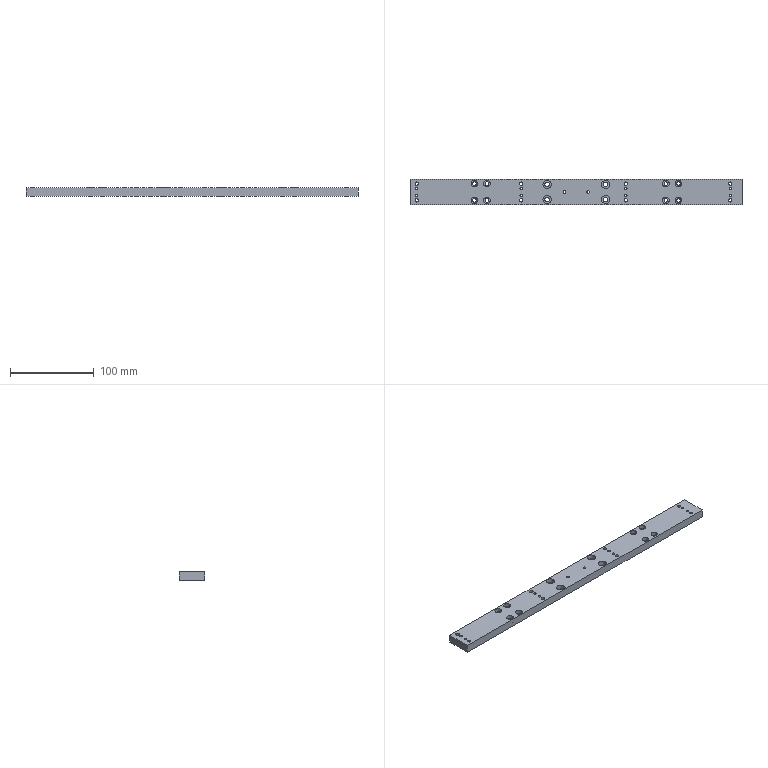Component | SolidWorks | JQ-2-0-003-1 | 1 solid | 102 faces | box 397 x 30 x 10 mm | volume 112652 mm3 | cylinder 84 | plane 18 | commonest cylinder face diameters 3 x20 8 x16 4.5 x16 4 x16 10 x8 5.5 x8
build123d program:
from build123d import *

# Parameters (mm, degrees)
SKETCH1_W                                            = 397
SKETCH1_H                                            = 30
BOSS_EXTRUDE1_DEPTH                                  = 10
HOLE_SIZE_ACCORDING_TO_TYPE_2_OF_HEX_SOC_D           = 5.5
HOLE_SIZE_ACCORDING_TO_TYPE_2_OF_HEX_SOC_CBORE_D     = 10
HOLE_SIZE_ACCORDING_TO_TYPE_2_OF_HEX_SOC_CBORE_DEPTH = 5.7
M4_TAPPED_HOLE1_D                                    = 4
HOLE_SIZE_ACCORDING_TO_TYPE_2_OF_HEX_2_D             = 4.5
HOLE_SIZE_ACCORDING_TO_TYPE_2_OF_HEX_2_CBORE_D       = 8
HOLE_SIZE_ACCORDING_TO_TYPE_2_OF_HEX_2_CBORE_DEPTH   = 4.6
SKETCH8_R                                            = 1.5
CUT_EXTRUDE1_DEPTH                                   = 399.257
SKETCH9_R                                            = 1.5
CUT_EXTRUDE2_DEPTH                                   = 399.257


with BuildPart() as part:
    # Sketch1 → Boss-Extrude1 (new body)
    with BuildSketch(Plane.XY):
        with Locations((198.5, 15)):
            Rectangle(SKETCH1_W, SKETCH1_H)
    extrude(amount=BOSS_EXTRUDE1_DEPTH)

    # Hole Size according to type 2 of hex soc (through all)
    with Locations(Plane.XY.offset(10)):
        with Locations((164, 24), (164, 6), (234, 6), (234, 24)):
            CounterBoreHole(HOLE_SIZE_ACCORDING_TO_TYPE_2_OF_HEX_SOC_D / 2, HOLE_SIZE_ACCORDING_TO_TYPE_2_OF_HEX_SOC_CBORE_D / 2, HOLE_SIZE_ACCORDING_TO_TYPE_2_OF_HEX_SOC_CBORE_DEPTH)

    # M4 Tapped Hole1 (through all)
    with Locations(Plane.XY.offset(10)):
        with Locations((133, 25), (133, 5), (258, 25), (258, 5), (383, 25), (383, 5), (8, 25), (8, 5)):
            Hole(M4_TAPPED_HOLE1_D / 2)

    # Hole Size according to type 2 of hex 2 (through all)
    with Locations(Plane.XY.offset(10)):
        with Locations((77, 5), (77, 25), (92, 25), (92, 5), (306, 5), (306, 25), (321, 25), (321, 5)):
            CounterBoreHole(HOLE_SIZE_ACCORDING_TO_TYPE_2_OF_HEX_2_D / 2, HOLE_SIZE_ACCORDING_TO_TYPE_2_OF_HEX_2_CBORE_D / 2, HOLE_SIZE_ACCORDING_TO_TYPE_2_OF_HEX_2_CBORE_DEPTH)

    # Sketch8 → Cut-Extrude1 (cut, through all)
    with BuildSketch(Plane.XY.offset(10)):
        with Locations((8, 19)):
            Circle(SKETCH8_R)
        with Locations((8, 11)):
            Circle(SKETCH8_R)
        with Locations((133, 19)):
            Circle(SKETCH8_R)
        with Locations((133, 11)):
            Circle(SKETCH8_R)
        with Locations((258, 19)):
            Circle(SKETCH8_R)
        with Locations((258, 11)):
            Circle(SKETCH8_R)
        with Locations((383, 19)):
            Circle(SKETCH8_R)
        with Locations((383, 11)):
            Circle(SKETCH8_R)
    extrude(amount=-CUT_EXTRUDE1_DEPTH, mode=Mode.SUBTRACT)

    # Sketch9 → Cut-Extrude2 (cut, through all)
    with BuildSketch(Plane.XY.offset(10)):
        with Locations((213, 15)):
            Circle(SKETCH9_R)
        with Locations((185, 15)):
            Circle(SKETCH9_R)
    extrude(amount=-CUT_EXTRUDE2_DEPTH, mode=Mode.SUBTRACT)


solid = part.part

# Placed as in the assembly
solid = solid.moved(Location((-461.058, 14.339, 107.131), (0, 0, 0)))